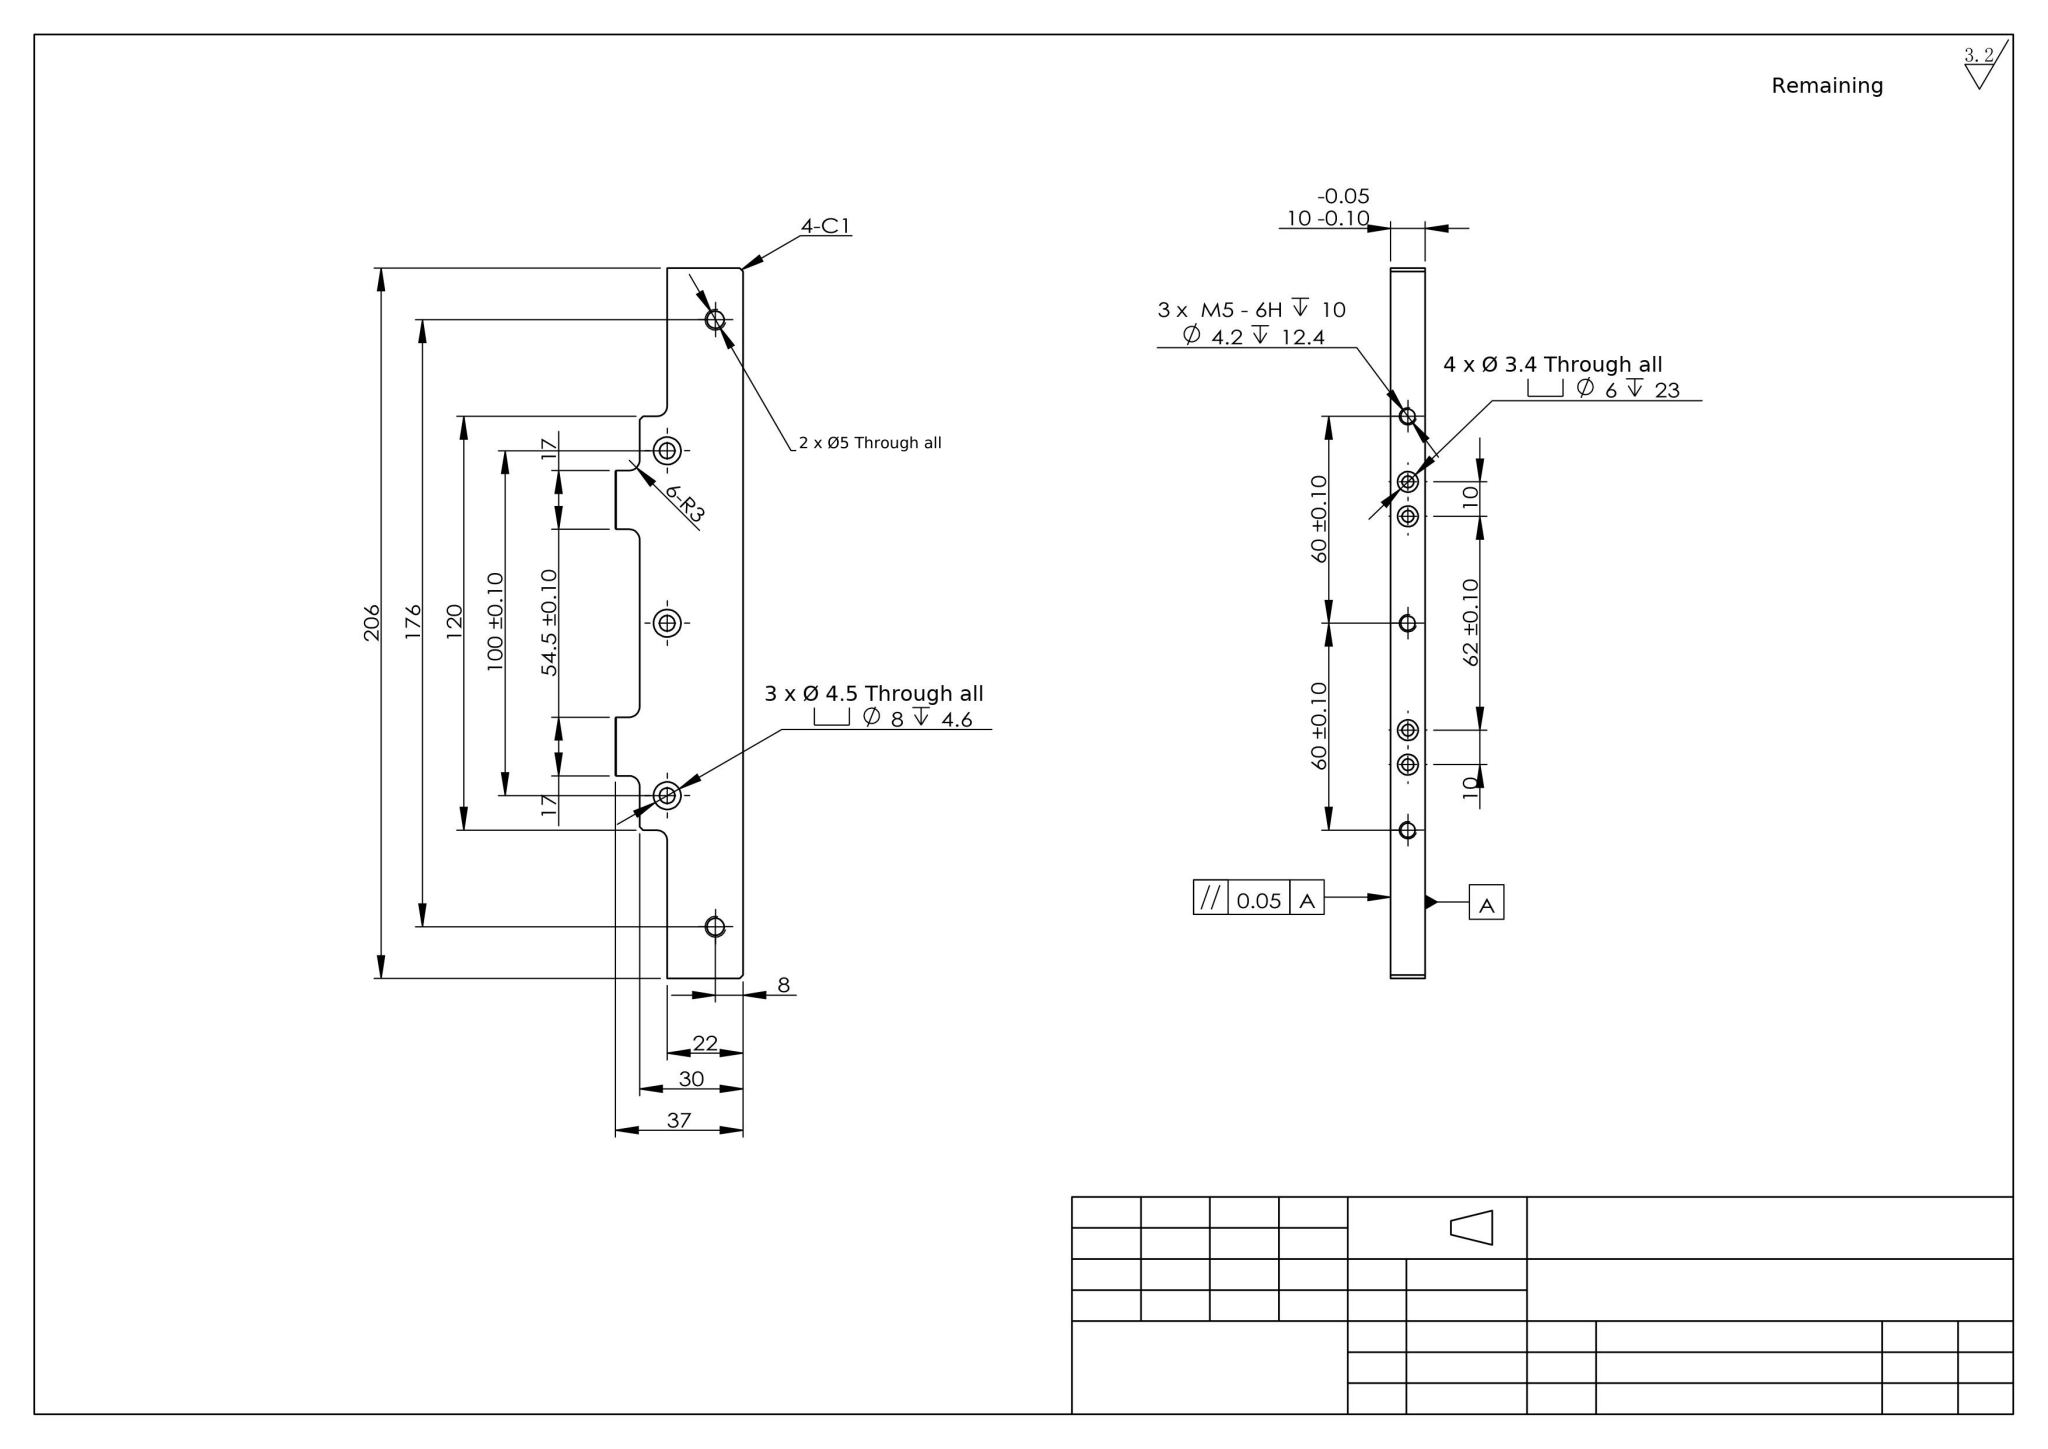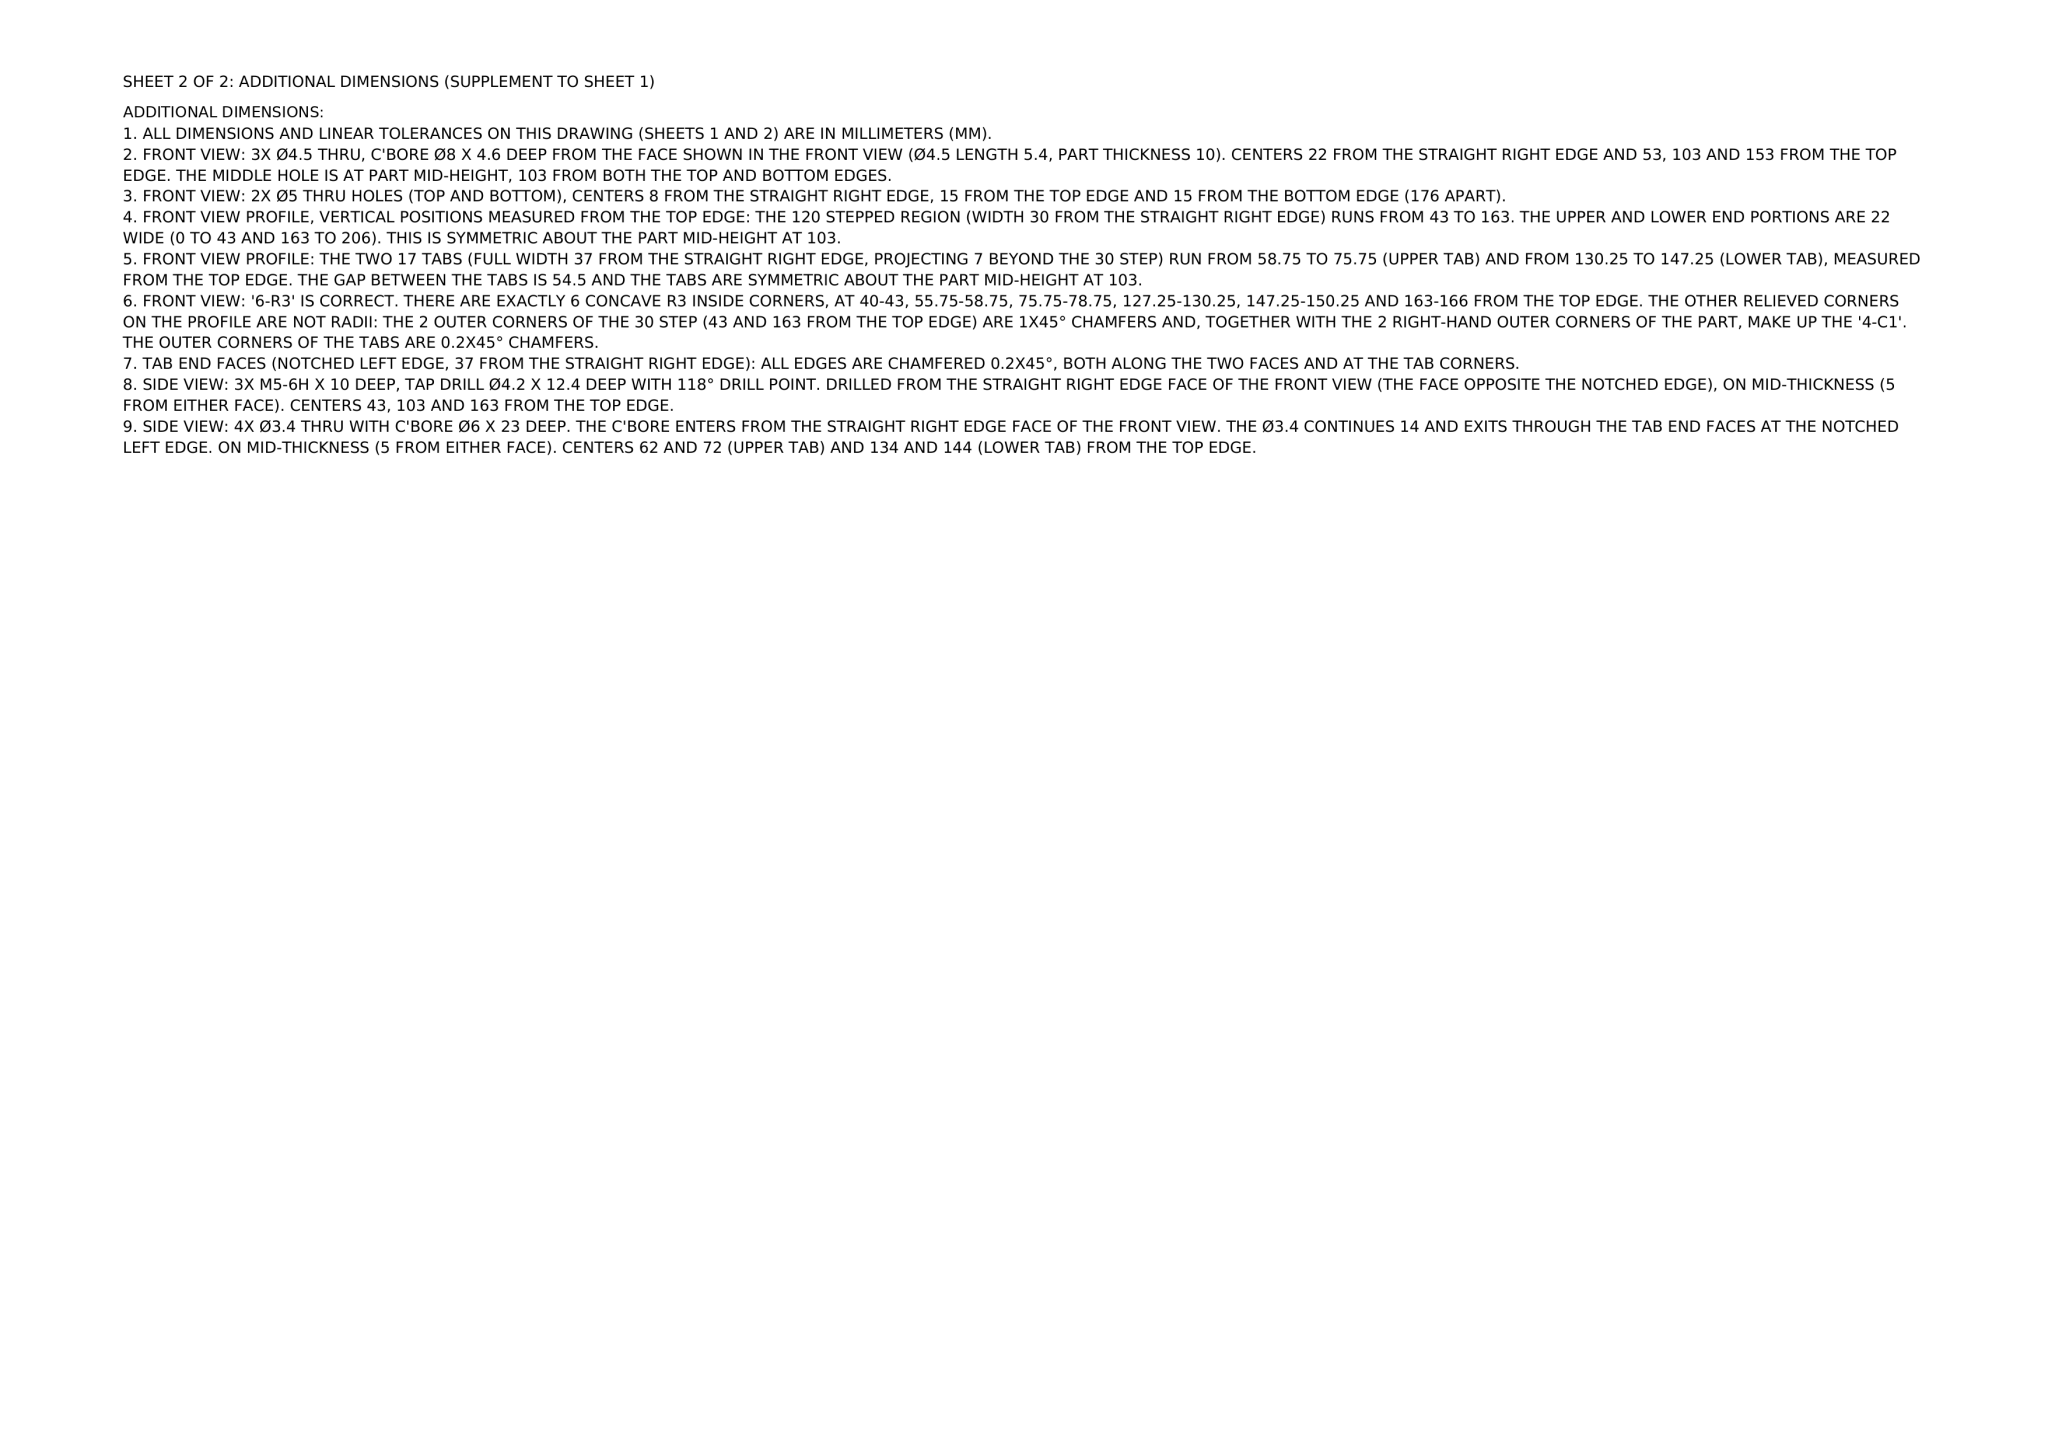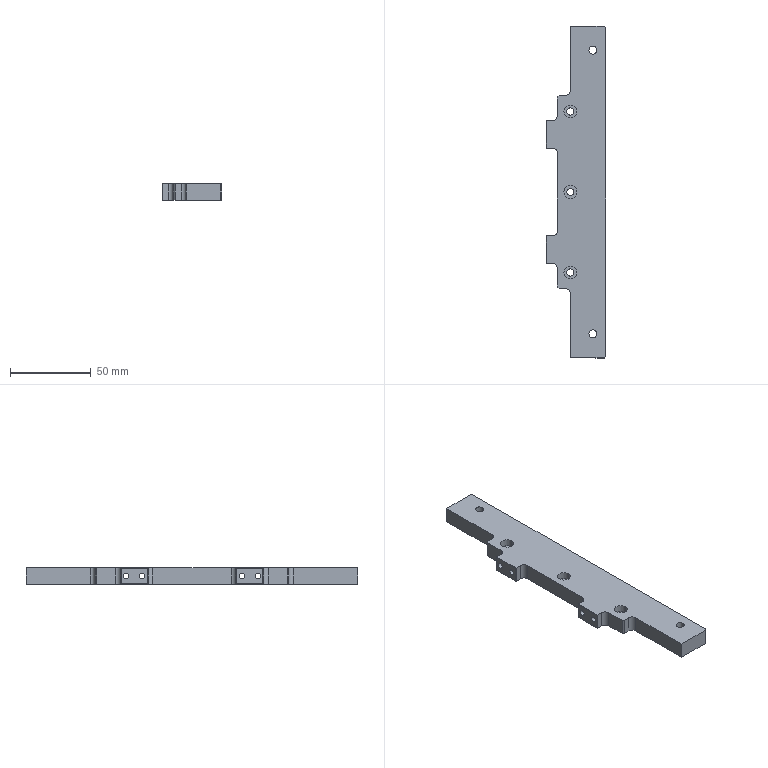Part | NX | mm | 1 solid | 87 faces | box 37 x 206 x 10 mm | volume 52407 mm3 | cylinder 44 | plane 37 | cone 6 | commonest cylinder face diameters 6 x14 3.4 x8 8 x6 4.5 x6 4.2 x6 5 x4